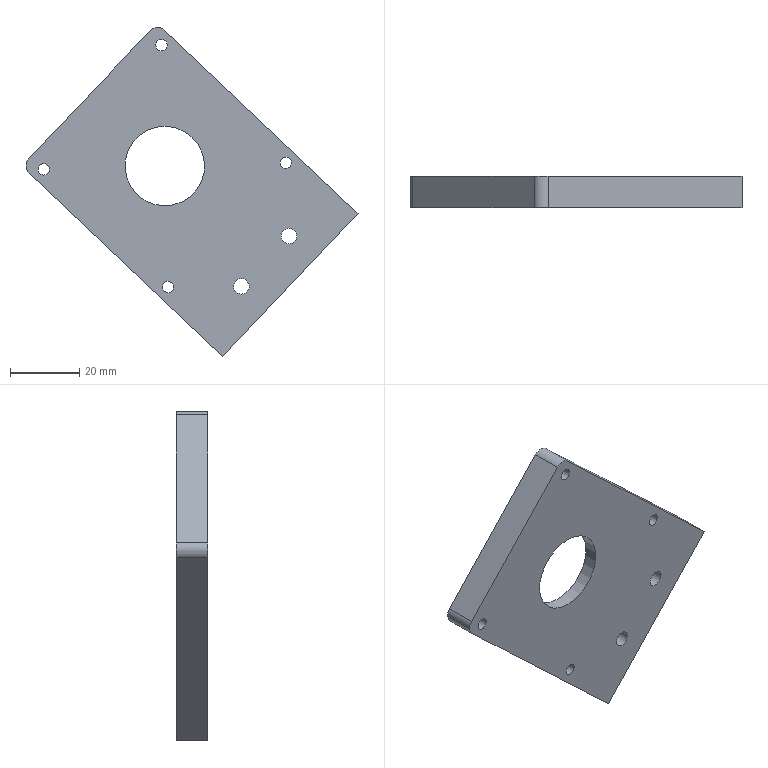Component | SolidWorks | 100-1_Copy(9)-1 | 1 solid | 31 faces | box 96.03 x 9 x 95.16 mm | volume 28622 mm3 | cylinder 22 | plane 9 | commonest cylinder face diameters 3.3 x8 8 x4 4.5 x4 50 x2 6 x2 23 x2
STEP:
#1=COLOUR_RGB('',0.7922,0.8196,0.9333);
#2=FILL_AREA_STYLE_COLOUR('',#1);
#3=FILL_AREA_STYLE('',(#2));
#4=SURFACE_STYLE_FILL_AREA(#3);
#5=SURFACE_SIDE_STYLE('',(#4));
#6=SURFACE_STYLE_USAGE(.BOTH.,#5);
#7=PRESENTATION_STYLE_ASSIGNMENT((#6));
#8=CARTESIAN_POINT('',(19.888,52.165,-78.736));
#9=VERTEX_POINT('',#8);
#10=CARTESIAN_POINT('',(19.265,52.165,-79.394));
#11=VERTEX_POINT('',#10);
#12=CARTESIAN_POINT('',(19.576,52.165,-79.065));
#13=DIRECTION('',(-0.,1.,0.));
#14=DIRECTION('',(-0.6879,0.,-0.7258));
#15=AXIS2_PLACEMENT_3D('',#12,#13,#14);
#16=CIRCLE('',#15,0.4528);
#17=EDGE_CURVE('',#9,#11,#16,.T.);
#18=ORIENTED_EDGE('',*,*,#17,.F.);
#19=CARTESIAN_POINT('',(19.576,52.165,-79.065));
#20=DIRECTION('',(-0.,1.,0.));
#21=DIRECTION('',(-0.6879,0.,-0.7258));
#22=AXIS2_PLACEMENT_3D('',#19,#20,#21);
#23=CIRCLE('',#22,0.4528);
#24=EDGE_CURVE('',#11,#9,#23,.T.);
#25=ORIENTED_EDGE('',*,*,#24,.F.);
#26=EDGE_LOOP('',(#18,#25));
#27=FACE_BOUND('',#26,.T.);
#28=CARTESIAN_POINT('',(18.899,52.165,-79.779));
#29=VERTEX_POINT('',#28);
#30=CARTESIAN_POINT('',(20.253,52.165,-78.351));
#31=VERTEX_POINT('',#30);
#32=CARTESIAN_POINT('',(19.576,52.165,-79.065));
#33=DIRECTION('',(-0.,1.,0.));
#34=DIRECTION('',(-0.6879,0.,-0.7258));
#35=AXIS2_PLACEMENT_3D('',#32,#33,#34);
#36=CIRCLE('',#35,0.9843);
#37=EDGE_CURVE('',#29,#31,#36,.T.);
#38=ORIENTED_EDGE('',*,*,#37,.T.);
#39=CARTESIAN_POINT('',(19.576,52.165,-79.065));
#40=DIRECTION('',(-0.,1.,0.));
#41=DIRECTION('',(-0.6879,0.,-0.7258));
#42=AXIS2_PLACEMENT_3D('',#39,#40,#41);
#43=CIRCLE('',#42,0.9843);
#44=EDGE_CURVE('',#31,#29,#43,.T.);
#45=ORIENTED_EDGE('',*,*,#44,.T.);
#46=EDGE_LOOP('',(#38,#45));
#47=FACE_OUTER_BOUND('',#46,.T.);
#48=CARTESIAN_POINT('',(19.576,52.165,-79.065));
#49=DIRECTION('',(-0.,1.,0.));
#50=DIRECTION('',(-0.6879,-0.,-0.7258));
#51=AXIS2_PLACEMENT_3D('',#48,#49,#50);
#52=PLANE('',#51);
#53=ADVANCED_FACE('',(#27,#47),#52,.T.);
#54=CARTESIAN_POINT('',(20.253,52.362,-78.351));
#55=VERTEX_POINT('',#54);
#56=CARTESIAN_POINT('',(20.253,52.165,-78.351));
#57=DIRECTION('',(-0.,1.,0.));
#58=VECTOR('',#57,39.37);
#59=LINE('',#56,#58);
#60=EDGE_CURVE('',#31,#55,#59,.T.);
#61=ORIENTED_EDGE('',*,*,#60,.F.);
#62=ORIENTED_EDGE('',*,*,#37,.F.);
#63=CARTESIAN_POINT('',(18.899,52.362,-79.779));
#64=VERTEX_POINT('',#63);
#65=CARTESIAN_POINT('',(18.899,52.165,-79.779));
#66=DIRECTION('',(-0.,1.,0.));
#67=VECTOR('',#66,39.37);
#68=LINE('',#65,#67);
#69=EDGE_CURVE('',#29,#64,#68,.T.);
#70=ORIENTED_EDGE('',*,*,#69,.T.);
#71=CARTESIAN_POINT('',(19.576,52.362,-79.065));
#72=DIRECTION('',(-0.,1.,0.));
#73=DIRECTION('',(-0.6879,0.,-0.7258));
#74=AXIS2_PLACEMENT_3D('',#71,#72,#73);
#75=CIRCLE('',#74,0.9843);
#76=EDGE_CURVE('',#64,#55,#75,.T.);
#77=ORIENTED_EDGE('',*,*,#76,.T.);
#78=EDGE_LOOP('',(#61,#62,#70,#77));
#79=FACE_OUTER_BOUND('',#78,.T.);
#80=CARTESIAN_POINT('',(19.576,52.165,-79.065));
#81=DIRECTION('',(-0.,1.,0.));
#82=DIRECTION('',(-0.6879,0.,-0.7258));
#83=AXIS2_PLACEMENT_3D('',#80,#81,#82);
#84=CYLINDRICAL_SURFACE('',#83,0.9843);
#85=ADVANCED_FACE('',(#79),#84,.F.);
#86=CARTESIAN_POINT('',(19.584,52.008,-77.64));
#87=VERTEX_POINT('',#86);
#88=CARTESIAN_POINT('',(19.584,52.362,-77.64));
#89=VERTEX_POINT('',#88);
#90=CARTESIAN_POINT('',(19.584,52.362,-77.64));
#91=DIRECTION('',(-0.,1.,0.));
#92=VECTOR('',#91,39.37);
#93=LINE('',#90,#92);
#94=EDGE_CURVE('',#87,#89,#93,.T.);
#95=ORIENTED_EDGE('',*,*,#94,.F.);
#96=CARTESIAN_POINT('',(19.494,52.008,-77.735));
#97=VERTEX_POINT('',#96);
#98=CARTESIAN_POINT('',(19.539,52.008,-77.687));
#99=DIRECTION('',(-0.,1.,0.));
#100=DIRECTION('',(-0.6879,0.,-0.7258));
#101=AXIS2_PLACEMENT_3D('',#98,#99,#100);
#102=CIRCLE('',#101,0.06496);
#103=EDGE_CURVE('',#97,#87,#102,.T.);
#104=ORIENTED_EDGE('',*,*,#103,.F.);
#105=CARTESIAN_POINT('',(19.494,52.362,-77.735));
#106=VERTEX_POINT('',#105);
#107=CARTESIAN_POINT('',(19.494,52.362,-77.735));
#108=DIRECTION('',(-0.,1.,0.));
#109=VECTOR('',#108,39.37);
#110=LINE('',#107,#109);
#111=EDGE_CURVE('',#97,#106,#110,.T.);
#112=ORIENTED_EDGE('',*,*,#111,.T.);
#113=CARTESIAN_POINT('',(19.539,52.362,-77.687));
#114=DIRECTION('',(-0.,1.,0.));
#115=DIRECTION('',(-0.6879,0.,-0.7258));
#116=AXIS2_PLACEMENT_3D('',#113,#114,#115);
#117=CIRCLE('',#116,0.06496);
#118=EDGE_CURVE('',#106,#89,#117,.T.);
#119=ORIENTED_EDGE('',*,*,#118,.T.);
#120=EDGE_LOOP('',(#95,#104,#112,#119));
#121=FACE_OUTER_BOUND('',#120,.T.);
#122=CARTESIAN_POINT('',(19.539,52.362,-77.687));
#123=DIRECTION('',(-0.,1.,0.));
#124=DIRECTION('',(-0.6879,0.,-0.7258));
#125=AXIS2_PLACEMENT_3D('',#122,#123,#124);
#126=CYLINDRICAL_SURFACE('',#125,0.06496);
#127=ADVANCED_FACE('',(#121),#126,.F.);
#128=CARTESIAN_POINT('',(18.243,52.008,-79.055));
#129=VERTEX_POINT('',#128);
#130=CARTESIAN_POINT('',(18.243,52.362,-79.055));
#131=VERTEX_POINT('',#130);
#132=CARTESIAN_POINT('',(18.243,52.362,-79.055));
#133=DIRECTION('',(-0.,1.,0.));
#134=VECTOR('',#133,39.37);
#135=LINE('',#132,#134);
#136=EDGE_CURVE('',#129,#131,#135,.T.);
#137=ORIENTED_EDGE('',*,*,#136,.F.);
#138=CARTESIAN_POINT('',(18.154,52.008,-79.149));
#139=VERTEX_POINT('',#138);
#140=CARTESIAN_POINT('',(18.199,52.008,-79.102));
#141=DIRECTION('',(-0.,1.,0.));
#142=DIRECTION('',(-0.6879,0.,-0.7258));
#143=AXIS2_PLACEMENT_3D('',#140,#141,#142);
#144=CIRCLE('',#143,0.06496);
#145=EDGE_CURVE('',#139,#129,#144,.T.);
#146=ORIENTED_EDGE('',*,*,#145,.F.);
#147=CARTESIAN_POINT('',(18.154,52.362,-79.149));
#148=VERTEX_POINT('',#147);
#149=CARTESIAN_POINT('',(18.154,52.362,-79.149));
#150=DIRECTION('',(-0.,1.,0.));
#151=VECTOR('',#150,39.37);
#152=LINE('',#149,#151);
#153=EDGE_CURVE('',#139,#148,#152,.T.);
#154=ORIENTED_EDGE('',*,*,#153,.T.);
#155=CARTESIAN_POINT('',(18.199,52.362,-79.102));
#156=DIRECTION('',(-0.,1.,0.));
#157=DIRECTION('',(-0.6879,0.,-0.7258));
#158=AXIS2_PLACEMENT_3D('',#155,#156,#157);
#159=CIRCLE('',#158,0.06496);
#160=EDGE_CURVE('',#148,#131,#159,.T.);
#161=ORIENTED_EDGE('',*,*,#160,.T.);
#162=EDGE_LOOP('',(#137,#146,#154,#161));
#163=FACE_OUTER_BOUND('',#162,.T.);
#164=CARTESIAN_POINT('',(18.199,52.362,-79.102));
#165=DIRECTION('',(-0.,1.,0.));
#166=DIRECTION('',(-0.6879,0.,-0.7258));
#167=AXIS2_PLACEMENT_3D('',#164,#165,#166);
#168=CYLINDRICAL_SURFACE('',#167,0.06496);
#169=ADVANCED_FACE('',(#163),#168,.F.);
#170=CARTESIAN_POINT('',(19.658,52.008,-80.395));
#171=VERTEX_POINT('',#170);
#172=CARTESIAN_POINT('',(19.658,52.362,-80.395));
#173=VERTEX_POINT('',#172);
#174=CARTESIAN_POINT('',(19.658,52.362,-80.395));
#175=DIRECTION('',(-0.,1.,0.));
#176=VECTOR('',#175,39.37);
#177=LINE('',#174,#176);
#178=EDGE_CURVE('',#171,#173,#177,.T.);
#179=ORIENTED_EDGE('',*,*,#178,.F.);
#180=CARTESIAN_POINT('',(19.568,52.008,-80.49));
#181=VERTEX_POINT('',#180);
#182=CARTESIAN_POINT('',(19.613,52.008,-80.442));
#183=DIRECTION('',(-0.,1.,0.));
#184=DIRECTION('',(-0.6879,0.,-0.7258));
#185=AXIS2_PLACEMENT_3D('',#182,#183,#184);
#186=CIRCLE('',#185,0.06496);
#187=EDGE_CURVE('',#181,#171,#186,.T.);
#188=ORIENTED_EDGE('',*,*,#187,.F.);
#189=CARTESIAN_POINT('',(19.568,52.362,-80.49));
#190=VERTEX_POINT('',#189);
#191=CARTESIAN_POINT('',(19.568,52.362,-80.49));
#192=DIRECTION('',(-0.,1.,0.));
#193=VECTOR('',#192,39.37);
#194=LINE('',#191,#193);
#195=EDGE_CURVE('',#181,#190,#194,.T.);
#196=ORIENTED_EDGE('',*,*,#195,.T.);
#197=CARTESIAN_POINT('',(19.613,52.362,-80.442));
#198=DIRECTION('',(-0.,1.,0.));
#199=DIRECTION('',(-0.6879,0.,-0.7258));
#200=AXIS2_PLACEMENT_3D('',#197,#198,#199);
#201=CIRCLE('',#200,0.06496);
#202=EDGE_CURVE('',#190,#173,#201,.T.);
#203=ORIENTED_EDGE('',*,*,#202,.T.);
#204=EDGE_LOOP('',(#179,#188,#196,#203));
#205=FACE_OUTER_BOUND('',#204,.T.);
#206=CARTESIAN_POINT('',(19.613,52.362,-80.442));
#207=DIRECTION('',(-0.,1.,0.));
#208=DIRECTION('',(-0.6879,0.,-0.7258));
#209=AXIS2_PLACEMENT_3D('',#206,#207,#208);
#210=CYLINDRICAL_SURFACE('',#209,0.06496);
#211=ADVANCED_FACE('',(#205),#210,.F.);
#212=CARTESIAN_POINT('',(20.998,52.008,-78.981));
#213=VERTEX_POINT('',#212);
#214=CARTESIAN_POINT('',(20.998,52.362,-78.981));
#215=VERTEX_POINT('',#214);
#216=CARTESIAN_POINT('',(20.998,52.362,-78.981));
#217=DIRECTION('',(-0.,1.,0.));
#218=VECTOR('',#217,39.37);
#219=LINE('',#216,#218);
#220=EDGE_CURVE('',#213,#215,#219,.T.);
#221=ORIENTED_EDGE('',*,*,#220,.F.);
#222=CARTESIAN_POINT('',(20.909,52.008,-79.075));
#223=VERTEX_POINT('',#222);
#224=CARTESIAN_POINT('',(20.954,52.008,-79.028));
#225=DIRECTION('',(-0.,1.,0.));
#226=DIRECTION('',(-0.6879,0.,-0.7258));
#227=AXIS2_PLACEMENT_3D('',#224,#225,#226);
#228=CIRCLE('',#227,0.06496);
#229=EDGE_CURVE('',#223,#213,#228,.T.);
#230=ORIENTED_EDGE('',*,*,#229,.F.);
#231=CARTESIAN_POINT('',(20.909,52.362,-79.075));
#232=VERTEX_POINT('',#231);
#233=CARTESIAN_POINT('',(20.909,52.362,-79.075));
#234=DIRECTION('',(-0.,1.,0.));
#235=VECTOR('',#234,39.37);
#236=LINE('',#233,#235);
#237=EDGE_CURVE('',#223,#232,#236,.T.);
#238=ORIENTED_EDGE('',*,*,#237,.T.);
#239=CARTESIAN_POINT('',(20.954,52.362,-79.028));
#240=DIRECTION('',(-0.,1.,0.));
#241=DIRECTION('',(-0.6879,0.,-0.7258));
#242=AXIS2_PLACEMENT_3D('',#239,#240,#241);
#243=CIRCLE('',#242,0.06496);
#244=EDGE_CURVE('',#232,#215,#243,.T.);
#245=ORIENTED_EDGE('',*,*,#244,.T.);
#246=EDGE_LOOP('',(#221,#230,#238,#245));
#247=FACE_OUTER_BOUND('',#246,.T.);
#248=CARTESIAN_POINT('',(20.954,52.362,-79.028));
#249=DIRECTION('',(-0.,1.,0.));
#250=DIRECTION('',(-0.6879,0.,-0.7258));
#251=AXIS2_PLACEMENT_3D('',#248,#249,#250);
#252=CYLINDRICAL_SURFACE('',#251,0.06496);
#253=ADVANCED_FACE('',(#247),#252,.F.);
#254=CARTESIAN_POINT('',(19.409,52.362,-77.524));
#255=VERTEX_POINT('',#254);
#256=CARTESIAN_POINT('',(19.576,52.362,-77.519));
#257=VERTEX_POINT('',#256);
#258=CARTESIAN_POINT('',(19.495,52.362,-77.605));
#259=DIRECTION('',(-0.,1.,0.));
#260=DIRECTION('',(0.6879,0.,0.7258));
#261=AXIS2_PLACEMENT_3D('',#258,#259,#260);
#262=CIRCLE('',#261,0.1181);
#263=EDGE_CURVE('',#255,#257,#262,.T.);
#264=ORIENTED_EDGE('',*,*,#263,.F.);
#265=CARTESIAN_POINT('',(19.409,52.008,-77.524));
#266=VERTEX_POINT('',#265);
#267=CARTESIAN_POINT('',(19.409,52.362,-77.524));
#268=DIRECTION('',(-0.,1.,0.));
#269=VECTOR('',#268,39.37);
#270=LINE('',#267,#269);
#271=EDGE_CURVE('',#266,#255,#270,.T.);
#272=ORIENTED_EDGE('',*,*,#271,.F.);
#273=CARTESIAN_POINT('',(19.576,52.008,-77.519));
#274=VERTEX_POINT('',#273);
#275=CARTESIAN_POINT('',(19.495,52.008,-77.605));
#276=DIRECTION('',(0.,-1.,-0.));
#277=DIRECTION('',(0.6879,0.,0.7258));
#278=AXIS2_PLACEMENT_3D('',#275,#276,#277);
#279=CIRCLE('',#278,0.1181);
#280=EDGE_CURVE('',#274,#266,#279,.T.);
#281=ORIENTED_EDGE('',*,*,#280,.F.);
#282=CARTESIAN_POINT('',(19.576,52.362,-77.519));
#283=DIRECTION('',(0.,-1.,-0.));
#284=VECTOR('',#283,39.37);
#285=LINE('',#282,#284);
#286=EDGE_CURVE('',#257,#274,#285,.T.);
#287=ORIENTED_EDGE('',*,*,#286,.F.);
#288=EDGE_LOOP('',(#264,#272,#281,#287));
#289=FACE_OUTER_BOUND('',#288,.T.);
#290=CARTESIAN_POINT('',(19.495,52.362,-77.605));
#291=DIRECTION('',(0.,-1.,-0.));
#292=DIRECTION('',(0.6879,0.,0.7258));
#293=AXIS2_PLACEMENT_3D('',#290,#291,#292);
#294=CYLINDRICAL_SURFACE('',#293,0.1181);
#295=ADVANCED_FACE('',(#289),#294,.T.);
#296=CARTESIAN_POINT('',(18.033,52.362,-79.148));
#297=VERTEX_POINT('',#296);
#298=CARTESIAN_POINT('',(18.028,52.362,-78.981));
#299=VERTEX_POINT('',#298);
#300=CARTESIAN_POINT('',(18.114,52.362,-79.062));
#301=DIRECTION('',(-0.,1.,0.));
#302=DIRECTION('',(0.6879,0.,0.7258));
#303=AXIS2_PLACEMENT_3D('',#300,#301,#302);
#304=CIRCLE('',#303,0.1181);
#305=EDGE_CURVE('',#297,#299,#304,.T.);
#306=ORIENTED_EDGE('',*,*,#305,.F.);
#307=CARTESIAN_POINT('',(18.033,52.008,-79.148));
#308=VERTEX_POINT('',#307);
#309=CARTESIAN_POINT('',(18.033,52.362,-79.148));
#310=DIRECTION('',(-0.,1.,0.));
#311=VECTOR('',#310,39.37);
#312=LINE('',#309,#311);
#313=EDGE_CURVE('',#308,#297,#312,.T.);
#314=ORIENTED_EDGE('',*,*,#313,.F.);
#315=CARTESIAN_POINT('',(18.028,52.008,-78.981));
#316=VERTEX_POINT('',#315);
#317=CARTESIAN_POINT('',(18.114,52.008,-79.062));
#318=DIRECTION('',(0.,-1.,-0.));
#319=DIRECTION('',(0.6879,0.,0.7258));
#320=AXIS2_PLACEMENT_3D('',#317,#318,#319);
#321=CIRCLE('',#320,0.1181);
#322=EDGE_CURVE('',#316,#308,#321,.T.);
#323=ORIENTED_EDGE('',*,*,#322,.F.);
#324=CARTESIAN_POINT('',(18.028,52.362,-78.981));
#325=DIRECTION('',(0.,-1.,-0.));
#326=VECTOR('',#325,39.37);
#327=LINE('',#324,#326);
#328=EDGE_CURVE('',#299,#316,#327,.T.);
#329=ORIENTED_EDGE('',*,*,#328,.F.);
#330=EDGE_LOOP('',(#306,#314,#323,#329));
#331=FACE_OUTER_BOUND('',#330,.T.);
#332=CARTESIAN_POINT('',(18.114,52.362,-79.062));
#333=DIRECTION('',(0.,-1.,-0.));
#334=DIRECTION('',(0.6879,0.,0.7258));
#335=AXIS2_PLACEMENT_3D('',#332,#333,#334);
#336=CYLINDRICAL_SURFACE('',#335,0.1181);
#337=ADVANCED_FACE('',(#331),#336,.T.);
#338=CARTESIAN_POINT('',(21.098,52.185,-79.748));
#339=VERTEX_POINT('',#338);
#340=CARTESIAN_POINT('',(21.098,52.362,-79.748));
#341=VERTEX_POINT('',#340);
#342=CARTESIAN_POINT('',(21.098,52.362,-79.748));
#343=DIRECTION('',(-0.,1.,0.));
#344=VECTOR('',#343,39.37);
#345=LINE('',#342,#344);
#346=EDGE_CURVE('',#339,#341,#345,.T.);
#347=ORIENTED_EDGE('',*,*,#346,.F.);
#348=CARTESIAN_POINT('',(20.882,52.185,-79.977));
#349=VERTEX_POINT('',#348);
#350=CARTESIAN_POINT('',(20.99,52.185,-79.862));
#351=DIRECTION('',(-0.,1.,0.));
#352=DIRECTION('',(-0.6879,0.,-0.7258));
#353=AXIS2_PLACEMENT_3D('',#350,#351,#352);
#354=CIRCLE('',#353,0.1575);
#355=EDGE_CURVE('',#349,#339,#354,.T.);
#356=ORIENTED_EDGE('',*,*,#355,.F.);
#357=CARTESIAN_POINT('',(20.882,52.362,-79.977));
#358=VERTEX_POINT('',#357);
#359=CARTESIAN_POINT('',(20.882,52.362,-79.977));
#360=DIRECTION('',(-0.,1.,0.));
#361=VECTOR('',#360,39.37);
#362=LINE('',#359,#361);
#363=EDGE_CURVE('',#349,#358,#362,.T.);
#364=ORIENTED_EDGE('',*,*,#363,.T.);
#365=CARTESIAN_POINT('',(20.99,52.362,-79.862));
#366=DIRECTION('',(-0.,1.,0.));
#367=DIRECTION('',(-0.6879,0.,-0.7258));
#368=AXIS2_PLACEMENT_3D('',#365,#366,#367);
#369=CIRCLE('',#368,0.1575);
#370=EDGE_CURVE('',#358,#341,#369,.T.);
#371=ORIENTED_EDGE('',*,*,#370,.T.);
#372=EDGE_LOOP('',(#347,#356,#364,#371));
#373=FACE_OUTER_BOUND('',#372,.T.);
#374=CARTESIAN_POINT('',(20.99,52.362,-79.862));
#375=DIRECTION('',(-0.,1.,0.));
#376=DIRECTION('',(-0.6879,0.,-0.7258));
#377=AXIS2_PLACEMENT_3D('',#374,#375,#376);
#378=CYLINDRICAL_SURFACE('',#377,0.1575);
#379=ADVANCED_FACE('',(#373),#378,.F.);
#380=CARTESIAN_POINT('',(20.929,52.185,-79.927));
#381=VERTEX_POINT('',#380);
#382=CARTESIAN_POINT('',(21.051,52.185,-79.798));
#383=VERTEX_POINT('',#382);
#384=CARTESIAN_POINT('',(20.99,52.185,-79.862));
#385=DIRECTION('',(-0.,1.,0.));
#386=DIRECTION('',(-0.6879,0.,-0.7258));
#387=AXIS2_PLACEMENT_3D('',#384,#385,#386);
#388=CIRCLE('',#387,0.08858);
#389=EDGE_CURVE('',#381,#383,#388,.T.);
#390=ORIENTED_EDGE('',*,*,#389,.F.);
#391=CARTESIAN_POINT('',(20.99,52.185,-79.862));
#392=DIRECTION('',(-0.,1.,0.));
#393=DIRECTION('',(-0.6879,0.,-0.7258));
#394=AXIS2_PLACEMENT_3D('',#391,#392,#393);
#395=CIRCLE('',#394,0.08858);
#396=EDGE_CURVE('',#383,#381,#395,.T.);
#397=ORIENTED_EDGE('',*,*,#396,.F.);
#398=EDGE_LOOP('',(#390,#397));
#399=FACE_BOUND('',#398,.T.);
#400=ORIENTED_EDGE('',*,*,#355,.T.);
#401=CARTESIAN_POINT('',(20.99,52.185,-79.862));
#402=DIRECTION('',(-0.,1.,0.));
#403=DIRECTION('',(-0.6879,0.,-0.7258));
#404=AXIS2_PLACEMENT_3D('',#401,#402,#403);
#405=CIRCLE('',#404,0.1575);
#406=EDGE_CURVE('',#339,#349,#405,.T.);
#407=ORIENTED_EDGE('',*,*,#406,.T.);
#408=EDGE_LOOP('',(#400,#407));
#409=FACE_OUTER_BOUND('',#408,.T.);
#410=CARTESIAN_POINT('',(20.929,52.185,-79.927));
#411=DIRECTION('',(0.,-1.,-0.));
#412=DIRECTION('',(0.7258,0.,-0.6879));
#413=AXIS2_PLACEMENT_3D('',#410,#411,#412);
#414=PLANE('',#413);
#415=ADVANCED_FACE('',(#399,#409),#414,.F.);
#416=CARTESIAN_POINT('',(21.051,52.008,-79.798));
#417=VERTEX_POINT('',#416);
#418=CARTESIAN_POINT('',(21.051,52.362,-79.798));
#419=DIRECTION('',(-0.,1.,0.));
#420=VECTOR('',#419,39.37);
#421=LINE('',#418,#420);
#422=EDGE_CURVE('',#417,#383,#421,.T.);
#423=ORIENTED_EDGE('',*,*,#422,.F.);
#424=CARTESIAN_POINT('',(20.929,52.008,-79.927));
#425=VERTEX_POINT('',#424);
#426=CARTESIAN_POINT('',(20.99,52.008,-79.862));
#427=DIRECTION('',(-0.,1.,0.));
#428=DIRECTION('',(-0.6879,0.,-0.7258));
#429=AXIS2_PLACEMENT_3D('',#426,#427,#428);
#430=CIRCLE('',#429,0.08858);
#431=EDGE_CURVE('',#425,#417,#430,.T.);
#432=ORIENTED_EDGE('',*,*,#431,.F.);
#433=CARTESIAN_POINT('',(20.929,52.362,-79.927));
#434=DIRECTION('',(-0.,1.,0.));
#435=VECTOR('',#434,39.37);
#436=LINE('',#433,#435);
#437=EDGE_CURVE('',#425,#381,#436,.T.);
#438=ORIENTED_EDGE('',*,*,#437,.T.);
#439=ORIENTED_EDGE('',*,*,#389,.T.);
#440=EDGE_LOOP('',(#423,#432,#438,#439));
#441=FACE_OUTER_BOUND('',#440,.T.);
#442=CARTESIAN_POINT('',(20.99,52.362,-79.862));
#443=DIRECTION('',(-0.,1.,0.));
#444=DIRECTION('',(-0.6879,0.,-0.7258));
#445=AXIS2_PLACEMENT_3D('',#442,#443,#444);
#446=CYLINDRICAL_SURFACE('',#445,0.08858);
#447=ADVANCED_FACE('',(#441),#446,.F.);
#448=CARTESIAN_POINT('',(20.557,52.185,-80.32));
#449=VERTEX_POINT('',#448);
#450=CARTESIAN_POINT('',(20.557,52.362,-80.32));
#451=VERTEX_POINT('',#450);
#452=CARTESIAN_POINT('',(20.557,52.362,-80.32));
#453=DIRECTION('',(-0.,1.,0.));
#454=VECTOR('',#453,39.37);
#455=LINE('',#452,#454);
#456=EDGE_CURVE('',#449,#451,#455,.T.);
#457=ORIENTED_EDGE('',*,*,#456,.F.);
#458=CARTESIAN_POINT('',(20.34,52.185,-80.548));
#459=VERTEX_POINT('',#458);
#460=CARTESIAN_POINT('',(20.448,52.185,-80.434));
#461=DIRECTION('',(-0.,1.,0.));
#462=DIRECTION('',(-0.6879,0.,-0.7258));
#463=AXIS2_PLACEMENT_3D('',#460,#461,#462);
#464=CIRCLE('',#463,0.1575);
#465=EDGE_CURVE('',#459,#449,#464,.T.);
#466=ORIENTED_EDGE('',*,*,#465,.F.);
#467=CARTESIAN_POINT('',(20.34,52.362,-80.548));
#468=VERTEX_POINT('',#467);
#469=CARTESIAN_POINT('',(20.34,52.362,-80.548));
#470=DIRECTION('',(-0.,1.,0.));
#471=VECTOR('',#470,39.37);
#472=LINE('',#469,#471);
#473=EDGE_CURVE('',#459,#468,#472,.T.);
#474=ORIENTED_EDGE('',*,*,#473,.T.);
#475=CARTESIAN_POINT('',(20.448,52.362,-80.434));
#476=DIRECTION('',(-0.,1.,0.));
#477=DIRECTION('',(-0.6879,0.,-0.7258));
#478=AXIS2_PLACEMENT_3D('',#475,#476,#477);
#479=CIRCLE('',#478,0.1575);
#480=EDGE_CURVE('',#468,#451,#479,.T.);
#481=ORIENTED_EDGE('',*,*,#480,.T.);
#482=EDGE_LOOP('',(#457,#466,#474,#481));
#483=FACE_OUTER_BOUND('',#482,.T.);
#484=CARTESIAN_POINT('',(20.448,52.362,-80.434));
#485=DIRECTION('',(-0.,1.,0.));
#486=DIRECTION('',(-0.6879,0.,-0.7258));
#487=AXIS2_PLACEMENT_3D('',#484,#485,#486);
#488=CYLINDRICAL_SURFACE('',#487,0.1575);
#489=ADVANCED_FACE('',(#483),#488,.F.);
#490=CARTESIAN_POINT('',(20.387,52.185,-80.498));
#491=VERTEX_POINT('',#490);
#492=CARTESIAN_POINT('',(20.509,52.185,-80.37));
#493=VERTEX_POINT('',#492);
#494=CARTESIAN_POINT('',(20.448,52.185,-80.434));
#495=DIRECTION('',(-0.,1.,0.));
#496=DIRECTION('',(-0.6879,0.,-0.7258));
#497=AXIS2_PLACEMENT_3D('',#494,#495,#496);
#498=CIRCLE('',#497,0.08858);
#499=EDGE_CURVE('',#491,#493,#498,.T.);
#500=ORIENTED_EDGE('',*,*,#499,.F.);
#501=CARTESIAN_POINT('',(20.448,52.185,-80.434));
#502=DIRECTION('',(-0.,1.,0.));
#503=DIRECTION('',(-0.6879,0.,-0.7258));
#504=AXIS2_PLACEMENT_3D('',#501,#502,#503);
#505=CIRCLE('',#504,0.08858);
#506=EDGE_CURVE('',#493,#491,#505,.T.);
#507=ORIENTED_EDGE('',*,*,#506,.F.);
#508=EDGE_LOOP('',(#500,#507));
#509=FACE_BOUND('',#508,.T.);
#510=ORIENTED_EDGE('',*,*,#465,.T.);
#511=CARTESIAN_POINT('',(20.448,52.185,-80.434));
#512=DIRECTION('',(-0.,1.,0.));
#513=DIRECTION('',(-0.6879,0.,-0.7258));
#514=AXIS2_PLACEMENT_3D('',#511,#512,#513);
#515=CIRCLE('',#514,0.1575);
#516=EDGE_CURVE('',#449,#459,#515,.T.);
#517=ORIENTED_EDGE('',*,*,#516,.T.);
#518=EDGE_LOOP('',(#510,#517));
#519=FACE_OUTER_BOUND('',#518,.T.);
#520=CARTESIAN_POINT('',(20.387,52.185,-80.498));
#521=DIRECTION('',(0.,-1.,-0.));
#522=DIRECTION('',(0.7258,0.,-0.6879));
#523=AXIS2_PLACEMENT_3D('',#520,#521,#522);
#524=PLANE('',#523);
#525=ADVANCED_FACE('',(#509,#519),#524,.F.);
#526=CARTESIAN_POINT('',(20.509,52.008,-80.37));
#527=VERTEX_POINT('',#526);
#528=CARTESIAN_POINT('',(20.509,52.362,-80.37));
#529=DIRECTION('',(-0.,1.,0.));
#530=VECTOR('',#529,39.37);
#531=LINE('',#528,#530);
#532=EDGE_CURVE('',#527,#493,#531,.T.);
#533=ORIENTED_EDGE('',*,*,#532,.F.);
#534=CARTESIAN_POINT('',(20.387,52.008,-80.498));
#535=VERTEX_POINT('',#534);
#536=CARTESIAN_POINT('',(20.448,52.008,-80.434));
#537=DIRECTION('',(-0.,1.,0.));
#538=DIRECTION('',(-0.6879,0.,-0.7258));
#539=AXIS2_PLACEMENT_3D('',#536,#537,#538);
#540=CIRCLE('',#539,0.08858);
#541=EDGE_CURVE('',#535,#527,#540,.T.);
#542=ORIENTED_EDGE('',*,*,#541,.F.);
#543=CARTESIAN_POINT('',(20.387,52.362,-80.498));
#544=DIRECTION('',(-0.,1.,0.));
#545=VECTOR('',#544,39.37);
#546=LINE('',#543,#545);
#547=EDGE_CURVE('',#535,#491,#546,.T.);
#548=ORIENTED_EDGE('',*,*,#547,.T.);
#549=ORIENTED_EDGE('',*,*,#499,.T.);
#550=EDGE_LOOP('',(#533,#542,#548,#549));
#551=FACE_OUTER_BOUND('',#550,.T.);
#552=CARTESIAN_POINT('',(20.448,52.362,-80.434));
#553=DIRECTION('',(-0.,1.,0.));
#554=DIRECTION('',(-0.6879,0.,-0.7258));
#555=AXIS2_PLACEMENT_3D('',#552,#553,#554);
#556=CYLINDRICAL_SURFACE('',#555,0.08858);
#557=ADVANCED_FACE('',(#551),#556,.F.);
#558=CARTESIAN_POINT('',(21.777,52.008,-79.605));
#559=VERTEX_POINT('',#558);
#560=CARTESIAN_POINT('',(20.233,52.008,-81.233));
#561=VERTEX_POINT('',#560);
#562=CARTESIAN_POINT('',(21.777,52.008,-79.605));
#563=DIRECTION('',(-0.6879,-0.,-0.7258));
#564=VECTOR('',#563,39.37);
#565=LINE('',#562,#564);
#566=EDGE_CURVE('',#559,#561,#565,.T.);
#567=ORIENTED_EDGE('',*,*,#566,.T.);
#568=CARTESIAN_POINT('',(20.233,52.362,-81.233));
#569=VERTEX_POINT('',#568);
#570=CARTESIAN_POINT('',(20.233,52.362,-81.233));
#571=DIRECTION('',(0.,-1.,-0.));
#572=VECTOR('',#571,39.37);
#573=LINE('',#570,#572);
#574=EDGE_CURVE('',#569,#561,#573,.T.);
#575=ORIENTED_EDGE('',*,*,#574,.F.);
#576=CARTESIAN_POINT('',(21.777,52.362,-79.605));
#577=VERTEX_POINT('',#576);
#578=CARTESIAN_POINT('',(21.777,52.362,-79.605));
#579=DIRECTION('',(-0.6879,-0.,-0.7258));
#580=VECTOR('',#579,39.37);
#581=LINE('',#578,#580);
#582=EDGE_CURVE('',#577,#569,#581,.T.);
#583=ORIENTED_EDGE('',*,*,#582,.F.);
#584=CARTESIAN_POINT('',(21.777,52.362,-79.605));
#585=DIRECTION('',(0.,-1.,-0.));
#586=VECTOR('',#585,39.37);
#587=LINE('',#584,#586);
#588=EDGE_CURVE('',#577,#559,#587,.T.);
#589=ORIENTED_EDGE('',*,*,#588,.T.);
#590=EDGE_LOOP('',(#567,#575,#583,#589));
#591=FACE_OUTER_BOUND('',#590,.T.);
#592=CARTESIAN_POINT('',(21.777,52.362,-79.605));
#593=DIRECTION('',(-0.7258,-0.,0.6879));
#594=DIRECTION('',(-0.6879,-0.,-0.7258));
#595=AXIS2_PLACEMENT_3D('',#592,#593,#594);
#596=PLANE('',#595);
#597=ADVANCED_FACE('',(#591),#596,.F.);
#598=CARTESIAN_POINT('',(21.777,52.362,-79.605));
#599=DIRECTION('',(0.7258,0.,-0.6879));
#600=VECTOR('',#599,39.37);
#601=LINE('',#598,#600);
#602=EDGE_CURVE('',#257,#577,#601,.T.);
#603=ORIENTED_EDGE('',*,*,#602,.F.);
#604=ORIENTED_EDGE('',*,*,#286,.T.);
#605=CARTESIAN_POINT('',(21.777,52.008,-79.605));
#606=DIRECTION('',(0.7258,0.,-0.6879));
#607=VECTOR('',#606,39.37);
#608=LINE('',#605,#607);
#609=EDGE_CURVE('',#274,#559,#608,.T.);
#610=ORIENTED_EDGE('',*,*,#609,.T.);
#611=ORIENTED_EDGE('',*,*,#588,.F.);
#612=EDGE_LOOP('',(#603,#604,#610,#611));
#613=FACE_OUTER_BOUND('',#612,.T.);
#614=CARTESIAN_POINT('',(21.777,52.362,-79.605));
#615=DIRECTION('',(-0.6879,-0.,-0.7258));
#616=DIRECTION('',(0.7258,0.,-0.6879));
#617=AXIS2_PLACEMENT_3D('',#614,#615,#616);
#618=PLANE('',#617);
#619=ADVANCED_FACE('',(#613),#618,.F.);
#620=CARTESIAN_POINT('',(19.491,52.362,-77.438));
#621=DIRECTION('',(0.6879,0.,0.7258));
#622=VECTOR('',#621,39.37);
#623=LINE('',#620,#622);
#624=EDGE_CURVE('',#299,#255,#623,.T.);
#625=ORIENTED_EDGE('',*,*,#624,.F.);
#626=ORIENTED_EDGE('',*,*,#328,.T.);
#627=CARTESIAN_POINT('',(19.491,52.008,-77.438));
#628=DIRECTION('',(0.6879,0.,0.7258));
#629=VECTOR('',#628,39.37);
#630=LINE('',#627,#629);
#631=EDGE_CURVE('',#316,#266,#630,.T.);
#632=ORIENTED_EDGE('',*,*,#631,.T.);
#633=ORIENTED_EDGE('',*,*,#271,.T.);
#634=EDGE_LOOP('',(#625,#626,#632,#633));
#635=FACE_OUTER_BOUND('',#634,.T.);
#636=CARTESIAN_POINT('',(19.491,52.362,-77.438));
#637=DIRECTION('',(0.7258,0.,-0.6879));
#638=DIRECTION('',(0.6879,0.,0.7258));
#639=AXIS2_PLACEMENT_3D('',#636,#637,#638);
#640=PLANE('',#639);
#641=ADVANCED_FACE('',(#635),#640,.F.);
#642=CARTESIAN_POINT('',(20.233,52.008,-81.233));
#643=DIRECTION('',(-0.7258,-0.,0.6879));
#644=VECTOR('',#643,39.37);
#645=LINE('',#642,#644);
#646=EDGE_CURVE('',#561,#308,#645,.T.);
#647=ORIENTED_EDGE('',*,*,#646,.T.);
#648=ORIENTED_EDGE('',*,*,#313,.T.);
#649=CARTESIAN_POINT('',(20.233,52.362,-81.233));
#650=DIRECTION('',(-0.7258,-0.,0.6879));
#651=VECTOR('',#650,39.37);
#652=LINE('',#649,#651);
#653=EDGE_CURVE('',#569,#297,#652,.T.);
#654=ORIENTED_EDGE('',*,*,#653,.F.);
#655=ORIENTED_EDGE('',*,*,#574,.T.);
#656=EDGE_LOOP('',(#647,#648,#654,#655));
#657=FACE_OUTER_BOUND('',#656,.T.);
#658=CARTESIAN_POINT('',(20.233,52.362,-81.233));
#659=DIRECTION('',(0.6879,0.,0.7258));
#660=DIRECTION('',(-0.,1.,0.));
#661=AXIS2_PLACEMENT_3D('',#658,#659,#660);
#662=PLANE('',#661);
#663=ADVANCED_FACE('',(#657),#662,.F.);
#664=CARTESIAN_POINT('',(19.888,52.008,-78.736));
#665=VERTEX_POINT('',#664);
#666=CARTESIAN_POINT('',(19.265,52.008,-79.394));
#667=VERTEX_POINT('',#666);
#668=CARTESIAN_POINT('',(19.576,52.008,-79.065));
#669=DIRECTION('',(-0.,1.,0.));
#670=DIRECTION('',(-0.6879,0.,-0.7258));
#671=AXIS2_PLACEMENT_3D('',#668,#669,#670);
#672=CIRCLE('',#671,0.4528);
#673=EDGE_CURVE('',#665,#667,#672,.T.);
#674=ORIENTED_EDGE('',*,*,#673,.T.);
#675=CARTESIAN_POINT('',(19.576,52.008,-79.065));
#676=DIRECTION('',(-0.,1.,0.));
#677=DIRECTION('',(-0.6879,0.,-0.7258));
#678=AXIS2_PLACEMENT_3D('',#675,#676,#677);
#679=CIRCLE('',#678,0.4528);
#680=EDGE_CURVE('',#667,#665,#679,.T.);
#681=ORIENTED_EDGE('',*,*,#680,.T.);
#682=EDGE_LOOP('',(#674,#681));
#683=FACE_BOUND('',#682,.T.);
#684=ORIENTED_EDGE('',*,*,#541,.T.);
#685=CARTESIAN_POINT('',(20.448,52.008,-80.434));
#686=DIRECTION('',(-0.,1.,0.));
#687=DIRECTION('',(-0.6879,0.,-0.7258));
#688=AXIS2_PLACEMENT_3D('',#685,#686,#687);
#689=CIRCLE('',#688,0.08858);
#690=EDGE_CURVE('',#527,#535,#689,.T.);
#691=ORIENTED_EDGE('',*,*,#690,.T.);
#692=EDGE_LOOP('',(#684,#691));
#693=FACE_BOUND('',#692,.T.);
#694=ORIENTED_EDGE('',*,*,#431,.T.);
#695=CARTESIAN_POINT('',(20.99,52.008,-79.862));
#696=DIRECTION('',(-0.,1.,0.));
#697=DIRECTION('',(-0.6879,0.,-0.7258));
#698=AXIS2_PLACEMENT_3D('',#695,#696,#697);
#699=CIRCLE('',#698,0.08858);
#700=EDGE_CURVE('',#417,#425,#699,.T.);
#701=ORIENTED_EDGE('',*,*,#700,.T.);
#702=EDGE_LOOP('',(#694,#701));
#703=FACE_BOUND('',#702,.T.);
#704=ORIENTED_EDGE('',*,*,#229,.T.);
#705=CARTESIAN_POINT('',(20.954,52.008,-79.028));
#706=DIRECTION('',(-0.,1.,0.));
#707=DIRECTION('',(-0.6879,0.,-0.7258));
#708=AXIS2_PLACEMENT_3D('',#705,#706,#707);
#709=CIRCLE('',#708,0.06496);
#710=EDGE_CURVE('',#213,#223,#709,.T.);
#711=ORIENTED_EDGE('',*,*,#710,.T.);
#712=EDGE_LOOP('',(#704,#711));
#713=FACE_BOUND('',#712,.T.);
#714=ORIENTED_EDGE('',*,*,#187,.T.);
#715=CARTESIAN_POINT('',(19.613,52.008,-80.442));
#716=DIRECTION('',(-0.,1.,0.));
#717=DIRECTION('',(-0.6879,0.,-0.7258));
#718=AXIS2_PLACEMENT_3D('',#715,#716,#717);
#719=CIRCLE('',#718,0.06496);
#720=EDGE_CURVE('',#171,#181,#719,.T.);
#721=ORIENTED_EDGE('',*,*,#720,.T.);
#722=EDGE_LOOP('',(#714,#721));
#723=FACE_BOUND('',#722,.T.);
#724=ORIENTED_EDGE('',*,*,#145,.T.);
#725=CARTESIAN_POINT('',(18.199,52.008,-79.102));
#726=DIRECTION('',(-0.,1.,0.));
#727=DIRECTION('',(-0.6879,0.,-0.7258));
#728=AXIS2_PLACEMENT_3D('',#725,#726,#727);
#729=CIRCLE('',#728,0.06496);
#730=EDGE_CURVE('',#129,#139,#729,.T.);
#731=ORIENTED_EDGE('',*,*,#730,.T.);
#732=EDGE_LOOP('',(#724,#731));
#733=FACE_BOUND('',#732,.T.);
#734=ORIENTED_EDGE('',*,*,#103,.T.);
#735=CARTESIAN_POINT('',(19.539,52.008,-77.687));
#736=DIRECTION('',(-0.,1.,0.));
#737=DIRECTION('',(-0.6879,0.,-0.7258));
#738=AXIS2_PLACEMENT_3D('',#735,#736,#737);
#739=CIRCLE('',#738,0.06496);
#740=EDGE_CURVE('',#87,#97,#739,.T.);
#741=ORIENTED_EDGE('',*,*,#740,.T.);
#742=EDGE_LOOP('',(#734,#741));
#743=FACE_BOUND('',#742,.T.);
#744=ORIENTED_EDGE('',*,*,#631,.F.);
#745=ORIENTED_EDGE('',*,*,#322,.T.);
#746=ORIENTED_EDGE('',*,*,#646,.F.);
#747=ORIENTED_EDGE('',*,*,#566,.F.);
#748=ORIENTED_EDGE('',*,*,#609,.F.);
#749=ORIENTED_EDGE('',*,*,#280,.T.);
#750=EDGE_LOOP('',(#744,#745,#746,#747,#748,#749));
#751=FACE_OUTER_BOUND('',#750,.T.);
#752=CARTESIAN_POINT('',(19.862,52.008,-79.336));
#753=DIRECTION('',(0.,-1.,-0.));
#754=DIRECTION('',(0.7258,0.,-0.6879));
#755=AXIS2_PLACEMENT_3D('',#752,#753,#754);
#756=PLANE('',#755);
#757=ADVANCED_FACE('',(#683,#693,#703,#713,#723,#733,#743,#751),#756,.T.);
#758=ORIENTED_EDGE('',*,*,#480,.F.);
#759=CARTESIAN_POINT('',(20.448,52.362,-80.434));
#760=DIRECTION('',(-0.,1.,0.));
#761=DIRECTION('',(-0.6879,0.,-0.7258));
#762=AXIS2_PLACEMENT_3D('',#759,#760,#761);
#763=CIRCLE('',#762,0.1575);
#764=EDGE_CURVE('',#451,#468,#763,.T.);
#765=ORIENTED_EDGE('',*,*,#764,.F.);
#766=EDGE_LOOP('',(#758,#765));
#767=FACE_BOUND('',#766,.T.);
#768=ORIENTED_EDGE('',*,*,#370,.F.);
#769=CARTESIAN_POINT('',(20.99,52.362,-79.862));
#770=DIRECTION('',(-0.,1.,0.));
#771=DIRECTION('',(-0.6879,0.,-0.7258));
#772=AXIS2_PLACEMENT_3D('',#769,#770,#771);
#773=CIRCLE('',#772,0.1575);
#774=EDGE_CURVE('',#341,#358,#773,.T.);
#775=ORIENTED_EDGE('',*,*,#774,.F.);
#776=EDGE_LOOP('',(#768,#775));
#777=FACE_BOUND('',#776,.T.);
#778=ORIENTED_EDGE('',*,*,#244,.F.);
#779=CARTESIAN_POINT('',(20.954,52.362,-79.028));
#780=DIRECTION('',(-0.,1.,0.));
#781=DIRECTION('',(-0.6879,0.,-0.7258));
#782=AXIS2_PLACEMENT_3D('',#779,#780,#781);
#783=CIRCLE('',#782,0.06496);
#784=EDGE_CURVE('',#215,#232,#783,.T.);
#785=ORIENTED_EDGE('',*,*,#784,.F.);
#786=EDGE_LOOP('',(#778,#785));
#787=FACE_BOUND('',#786,.T.);
#788=ORIENTED_EDGE('',*,*,#202,.F.);
#789=CARTESIAN_POINT('',(19.613,52.362,-80.442));
#790=DIRECTION('',(-0.,1.,0.));
#791=DIRECTION('',(-0.6879,0.,-0.7258));
#792=AXIS2_PLACEMENT_3D('',#789,#790,#791);
#793=CIRCLE('',#792,0.06496);
#794=EDGE_CURVE('',#173,#190,#793,.T.);
#795=ORIENTED_EDGE('',*,*,#794,.F.);
#796=EDGE_LOOP('',(#788,#795));
#797=FACE_BOUND('',#796,.T.);
#798=ORIENTED_EDGE('',*,*,#160,.F.);
#799=CARTESIAN_POINT('',(18.199,52.362,-79.102));
#800=DIRECTION('',(-0.,1.,0.));
#801=DIRECTION('',(-0.6879,0.,-0.7258));
#802=AXIS2_PLACEMENT_3D('',#799,#800,#801);
#803=CIRCLE('',#802,0.06496);
#804=EDGE_CURVE('',#131,#148,#803,.T.);
#805=ORIENTED_EDGE('',*,*,#804,.F.);
#806=EDGE_LOOP('',(#798,#805));
#807=FACE_BOUND('',#806,.T.);
#808=ORIENTED_EDGE('',*,*,#118,.F.);
#809=CARTESIAN_POINT('',(19.539,52.362,-77.687));
#810=DIRECTION('',(-0.,1.,0.));
#811=DIRECTION('',(-0.6879,0.,-0.7258));
#812=AXIS2_PLACEMENT_3D('',#809,#810,#811);
#813=CIRCLE('',#812,0.06496);
#814=EDGE_CURVE('',#89,#106,#813,.T.);
#815=ORIENTED_EDGE('',*,*,#814,.F.);
#816=EDGE_LOOP('',(#808,#815));
#817=FACE_BOUND('',#816,.T.);
#818=ORIENTED_EDGE('',*,*,#76,.F.);
#819=CARTESIAN_POINT('',(19.576,52.362,-79.065));
#820=DIRECTION('',(-0.,1.,0.));
#821=DIRECTION('',(-0.6879,0.,-0.7258));
#822=AXIS2_PLACEMENT_3D('',#819,#820,#821);
#823=CIRCLE('',#822,0.9843);
#824=EDGE_CURVE('',#55,#64,#823,.T.);
#825=ORIENTED_EDGE('',*,*,#824,.F.);
#826=EDGE_LOOP('',(#818,#825));
#827=FACE_BOUND('',#826,.T.);
#828=ORIENTED_EDGE('',*,*,#653,.T.);
#829=ORIENTED_EDGE('',*,*,#305,.T.);
#830=ORIENTED_EDGE('',*,*,#624,.T.);
#831=ORIENTED_EDGE('',*,*,#263,.T.);
#832=ORIENTED_EDGE('',*,*,#602,.T.);
#833=ORIENTED_EDGE('',*,*,#582,.T.);
#834=EDGE_LOOP('',(#828,#829,#830,#831,#832,#833));
#835=FACE_OUTER_BOUND('',#834,.T.);
#836=CARTESIAN_POINT('',(19.862,52.362,-79.336));
#837=DIRECTION('',(0.,-1.,-0.));
#838=DIRECTION('',(0.7258,0.,-0.6879));
#839=AXIS2_PLACEMENT_3D('',#836,#837,#838);
#840=PLANE('',#839);
#841=ADVANCED_FACE('',(#767,#777,#787,#797,#807,#817,#827,#835),#840,.F.);
#842=CARTESIAN_POINT('',(19.265,52.362,-79.394));
#843=DIRECTION('',(0.,-1.,-0.));
#844=VECTOR('',#843,39.37);
#845=LINE('',#842,#844);
#846=EDGE_CURVE('',#11,#667,#845,.T.);
#847=ORIENTED_EDGE('',*,*,#846,.F.);
#848=ORIENTED_EDGE('',*,*,#24,.T.);
#849=CARTESIAN_POINT('',(19.888,52.362,-78.736));
#850=DIRECTION('',(0.,-1.,-0.));
#851=VECTOR('',#850,39.37);
#852=LINE('',#849,#851);
#853=EDGE_CURVE('',#9,#665,#852,.T.);
#854=ORIENTED_EDGE('',*,*,#853,.T.);
#855=ORIENTED_EDGE('',*,*,#680,.F.);
#856=EDGE_LOOP('',(#847,#848,#854,#855));
#857=FACE_OUTER_BOUND('',#856,.T.);
#858=CARTESIAN_POINT('',(19.576,52.362,-79.065));
#859=DIRECTION('',(0.,-1.,-0.));
#860=DIRECTION('',(0.6879,0.,0.7258));
#861=AXIS2_PLACEMENT_3D('',#858,#859,#860);
#862=CYLINDRICAL_SURFACE('',#861,0.4528);
#863=ADVANCED_FACE('',(#857),#862,.F.);
#864=ORIENTED_EDGE('',*,*,#17,.T.);
#865=ORIENTED_EDGE('',*,*,#846,.T.);
#866=ORIENTED_EDGE('',*,*,#673,.F.);
#867=ORIENTED_EDGE('',*,*,#853,.F.);
#868=EDGE_LOOP('',(#864,#865,#866,#867));
#869=FACE_OUTER_BOUND('',#868,.T.);
#870=CARTESIAN_POINT('',(19.576,52.362,-79.065));
#871=DIRECTION('',(0.,-1.,-0.));
#872=DIRECTION('',(0.6879,0.,0.7258));
#873=AXIS2_PLACEMENT_3D('',#870,#871,#872);
#874=CYLINDRICAL_SURFACE('',#873,0.4528);
#875=ADVANCED_FACE('',(#869),#874,.F.);
#876=ORIENTED_EDGE('',*,*,#690,.F.);
#877=ORIENTED_EDGE('',*,*,#532,.T.);
#878=ORIENTED_EDGE('',*,*,#506,.T.);
#879=ORIENTED_EDGE('',*,*,#547,.F.);
#880=EDGE_LOOP('',(#876,#877,#878,#879));
#881=FACE_OUTER_BOUND('',#880,.T.);
#882=CARTESIAN_POINT('',(20.448,52.362,-80.434));
#883=DIRECTION('',(-0.,1.,0.));
#884=DIRECTION('',(-0.6879,0.,-0.7258));
#885=AXIS2_PLACEMENT_3D('',#882,#883,#884);
#886=CYLINDRICAL_SURFACE('',#885,0.08858);
#887=ADVANCED_FACE('',(#881),#886,.F.);
#888=ORIENTED_EDGE('',*,*,#516,.F.);
#889=ORIENTED_EDGE('',*,*,#456,.T.);
#890=ORIENTED_EDGE('',*,*,#764,.T.);
#891=ORIENTED_EDGE('',*,*,#473,.F.);
#892=EDGE_LOOP('',(#888,#889,#890,#891));
#893=FACE_OUTER_BOUND('',#892,.T.);
#894=CARTESIAN_POINT('',(20.448,52.362,-80.434));
#895=DIRECTION('',(-0.,1.,0.));
#896=DIRECTION('',(-0.6879,0.,-0.7258));
#897=AXIS2_PLACEMENT_3D('',#894,#895,#896);
#898=CYLINDRICAL_SURFACE('',#897,0.1575);
#899=ADVANCED_FACE('',(#893),#898,.F.);
#900=ORIENTED_EDGE('',*,*,#700,.F.);
#901=ORIENTED_EDGE('',*,*,#422,.T.);
#902=ORIENTED_EDGE('',*,*,#396,.T.);
#903=ORIENTED_EDGE('',*,*,#437,.F.);
#904=EDGE_LOOP('',(#900,#901,#902,#903));
#905=FACE_OUTER_BOUND('',#904,.T.);
#906=CARTESIAN_POINT('',(20.99,52.362,-79.862));
#907=DIRECTION('',(-0.,1.,0.));
#908=DIRECTION('',(-0.6879,0.,-0.7258));
#909=AXIS2_PLACEMENT_3D('',#906,#907,#908);
#910=CYLINDRICAL_SURFACE('',#909,0.08858);
#911=ADVANCED_FACE('',(#905),#910,.F.);
#912=ORIENTED_EDGE('',*,*,#406,.F.);
#913=ORIENTED_EDGE('',*,*,#346,.T.);
#914=ORIENTED_EDGE('',*,*,#774,.T.);
#915=ORIENTED_EDGE('',*,*,#363,.F.);
#916=EDGE_LOOP('',(#912,#913,#914,#915));
#917=FACE_OUTER_BOUND('',#916,.T.);
#918=CARTESIAN_POINT('',(20.99,52.362,-79.862));
#919=DIRECTION('',(-0.,1.,0.));
#920=DIRECTION('',(-0.6879,0.,-0.7258));
#921=AXIS2_PLACEMENT_3D('',#918,#919,#920);
#922=CYLINDRICAL_SURFACE('',#921,0.1575);
#923=ADVANCED_FACE('',(#917),#922,.F.);
#924=ORIENTED_EDGE('',*,*,#710,.F.);
#925=ORIENTED_EDGE('',*,*,#220,.T.);
#926=ORIENTED_EDGE('',*,*,#784,.T.);
#927=ORIENTED_EDGE('',*,*,#237,.F.);
#928=EDGE_LOOP('',(#924,#925,#926,#927));
#929=FACE_OUTER_BOUND('',#928,.T.);
#930=CARTESIAN_POINT('',(20.954,52.362,-79.028));
#931=DIRECTION('',(-0.,1.,0.));
#932=DIRECTION('',(-0.6879,0.,-0.7258));
#933=AXIS2_PLACEMENT_3D('',#930,#931,#932);
#934=CYLINDRICAL_SURFACE('',#933,0.06496);
#935=ADVANCED_FACE('',(#929),#934,.F.);
#936=ORIENTED_EDGE('',*,*,#720,.F.);
#937=ORIENTED_EDGE('',*,*,#178,.T.);
#938=ORIENTED_EDGE('',*,*,#794,.T.);
#939=ORIENTED_EDGE('',*,*,#195,.F.);
#940=EDGE_LOOP('',(#936,#937,#938,#939));
#941=FACE_OUTER_BOUND('',#940,.T.);
#942=CARTESIAN_POINT('',(19.613,52.362,-80.442));
#943=DIRECTION('',(-0.,1.,0.));
#944=DIRECTION('',(-0.6879,0.,-0.7258));
#945=AXIS2_PLACEMENT_3D('',#942,#943,#944);
#946=CYLINDRICAL_SURFACE('',#945,0.06496);
#947=ADVANCED_FACE('',(#941),#946,.F.);
#948=ORIENTED_EDGE('',*,*,#730,.F.);
#949=ORIENTED_EDGE('',*,*,#136,.T.);
#950=ORIENTED_EDGE('',*,*,#804,.T.);
#951=ORIENTED_EDGE('',*,*,#153,.F.);
#952=EDGE_LOOP('',(#948,#949,#950,#951));
#953=FACE_OUTER_BOUND('',#952,.T.);
#954=CARTESIAN_POINT('',(18.199,52.362,-79.102));
#955=DIRECTION('',(-0.,1.,0.));
#956=DIRECTION('',(-0.6879,0.,-0.7258));
#957=AXIS2_PLACEMENT_3D('',#954,#955,#956);
#958=CYLINDRICAL_SURFACE('',#957,0.06496);
#959=ADVANCED_FACE('',(#953),#958,.F.);
#960=ORIENTED_EDGE('',*,*,#740,.F.);
#961=ORIENTED_EDGE('',*,*,#94,.T.);
#962=ORIENTED_EDGE('',*,*,#814,.T.);
#963=ORIENTED_EDGE('',*,*,#111,.F.);
#964=EDGE_LOOP('',(#960,#961,#962,#963));
#965=FACE_OUTER_BOUND('',#964,.T.);
#966=CARTESIAN_POINT('',(19.539,52.362,-77.687));
#967=DIRECTION('',(-0.,1.,0.));
#968=DIRECTION('',(-0.6879,0.,-0.7258));
#969=AXIS2_PLACEMENT_3D('',#966,#967,#968);
#970=CYLINDRICAL_SURFACE('',#969,0.06496);
#971=ADVANCED_FACE('',(#965),#970,.F.);
#972=ORIENTED_EDGE('',*,*,#44,.F.);
#973=ORIENTED_EDGE('',*,*,#60,.T.);
#974=ORIENTED_EDGE('',*,*,#824,.T.);
#975=ORIENTED_EDGE('',*,*,#69,.F.);
#976=EDGE_LOOP('',(#972,#973,#974,#975));
#977=FACE_OUTER_BOUND('',#976,.T.);
#978=CARTESIAN_POINT('',(19.576,52.165,-79.065));
#979=DIRECTION('',(-0.,1.,0.));
#980=DIRECTION('',(-0.6879,0.,-0.7258));
#981=AXIS2_PLACEMENT_3D('',#978,#979,#980);
#982=CYLINDRICAL_SURFACE('',#981,0.9843);
#983=ADVANCED_FACE('',(#977),#982,.F.);
#984=CLOSED_SHELL('',(#53,#85,#127,#169,#211,#253,#295,#337,#379,#415,#447,#489,#525,#557,#597,#619,#641,#663,#757,#841,#863,#875,#887,#899,#911,#923,#935,#947,#959,#971,#983));
#985=MANIFOLD_SOLID_BREP('',#984);
#986=STYLED_ITEM('',(#7),#985);
#987=PRESENTATION_LAYER_ASSIGNMENT('','',(#986));
#988=CARTESIAN_POINT('',(0.,0.,0.));
#989=DIRECTION('',(0.,0.,1.));
#990=DIRECTION('',(1.,0.,0.));
#991=AXIS2_PLACEMENT_3D('',#988,#989,#990);
#992=(LENGTH_UNIT()NAMED_UNIT(*)SI_UNIT($,.METRE.));
#993=LENGTH_MEASURE_WITH_UNIT(LENGTH_MEASURE(0.0254),#992);
#994=DIMENSIONAL_EXPONENTS(1.,0.,0.,0.,0.,0.,0.);
#995=(CONVERSION_BASED_UNIT('',#993)LENGTH_UNIT()NAMED_UNIT(#994));
#996=UNCERTAINTY_MEASURE_WITH_UNIT(LENGTH_MEASURE(0.00001),#995,'','');
#997=(NAMED_UNIT(*)PLANE_ANGLE_UNIT()SI_UNIT($,.RADIAN.));
#998=(NAMED_UNIT(*)SI_UNIT($,.STERADIAN.)SOLID_ANGLE_UNIT());
#999=(GEOMETRIC_REPRESENTATION_CONTEXT(3)GLOBAL_UNCERTAINTY_ASSIGNED_CONTEXT((#996))GLOBAL_UNIT_ASSIGNED_CONTEXT((#995,#997,#998))REPRESENTATION_CONTEXT('',''));
#1000=ADVANCED_BREP_SHAPE_REPRESENTATION('',(#985,#991),#999);
#1001=(LENGTH_UNIT()NAMED_UNIT(*)SI_UNIT($,.METRE.));
#1002=LENGTH_MEASURE_WITH_UNIT(LENGTH_MEASURE(0.0254),#1001);
#1003=DIMENSIONAL_EXPONENTS(1.,0.,0.,0.,0.,0.,0.);
#1004=(CONVERSION_BASED_UNIT('',#1002)LENGTH_UNIT()NAMED_UNIT(#1003));
#1005=UNCERTAINTY_MEASURE_WITH_UNIT(LENGTH_MEASURE(0.00001),#1004,'','');
#1006=(NAMED_UNIT(*)PLANE_ANGLE_UNIT()SI_UNIT($,.RADIAN.));
#1007=(NAMED_UNIT(*)SI_UNIT($,.STERADIAN.)SOLID_ANGLE_UNIT());
#1008=(GEOMETRIC_REPRESENTATION_CONTEXT(3)GLOBAL_UNCERTAINTY_ASSIGNED_CONTEXT((#1005))GLOBAL_UNIT_ASSIGNED_CONTEXT((#1004,#1006,#1007))REPRESENTATION_CONTEXT('',''));
#1009=MECHANICAL_DESIGN_GEOMETRIC_PRESENTATION_REPRESENTATION('',(#986),#1008);